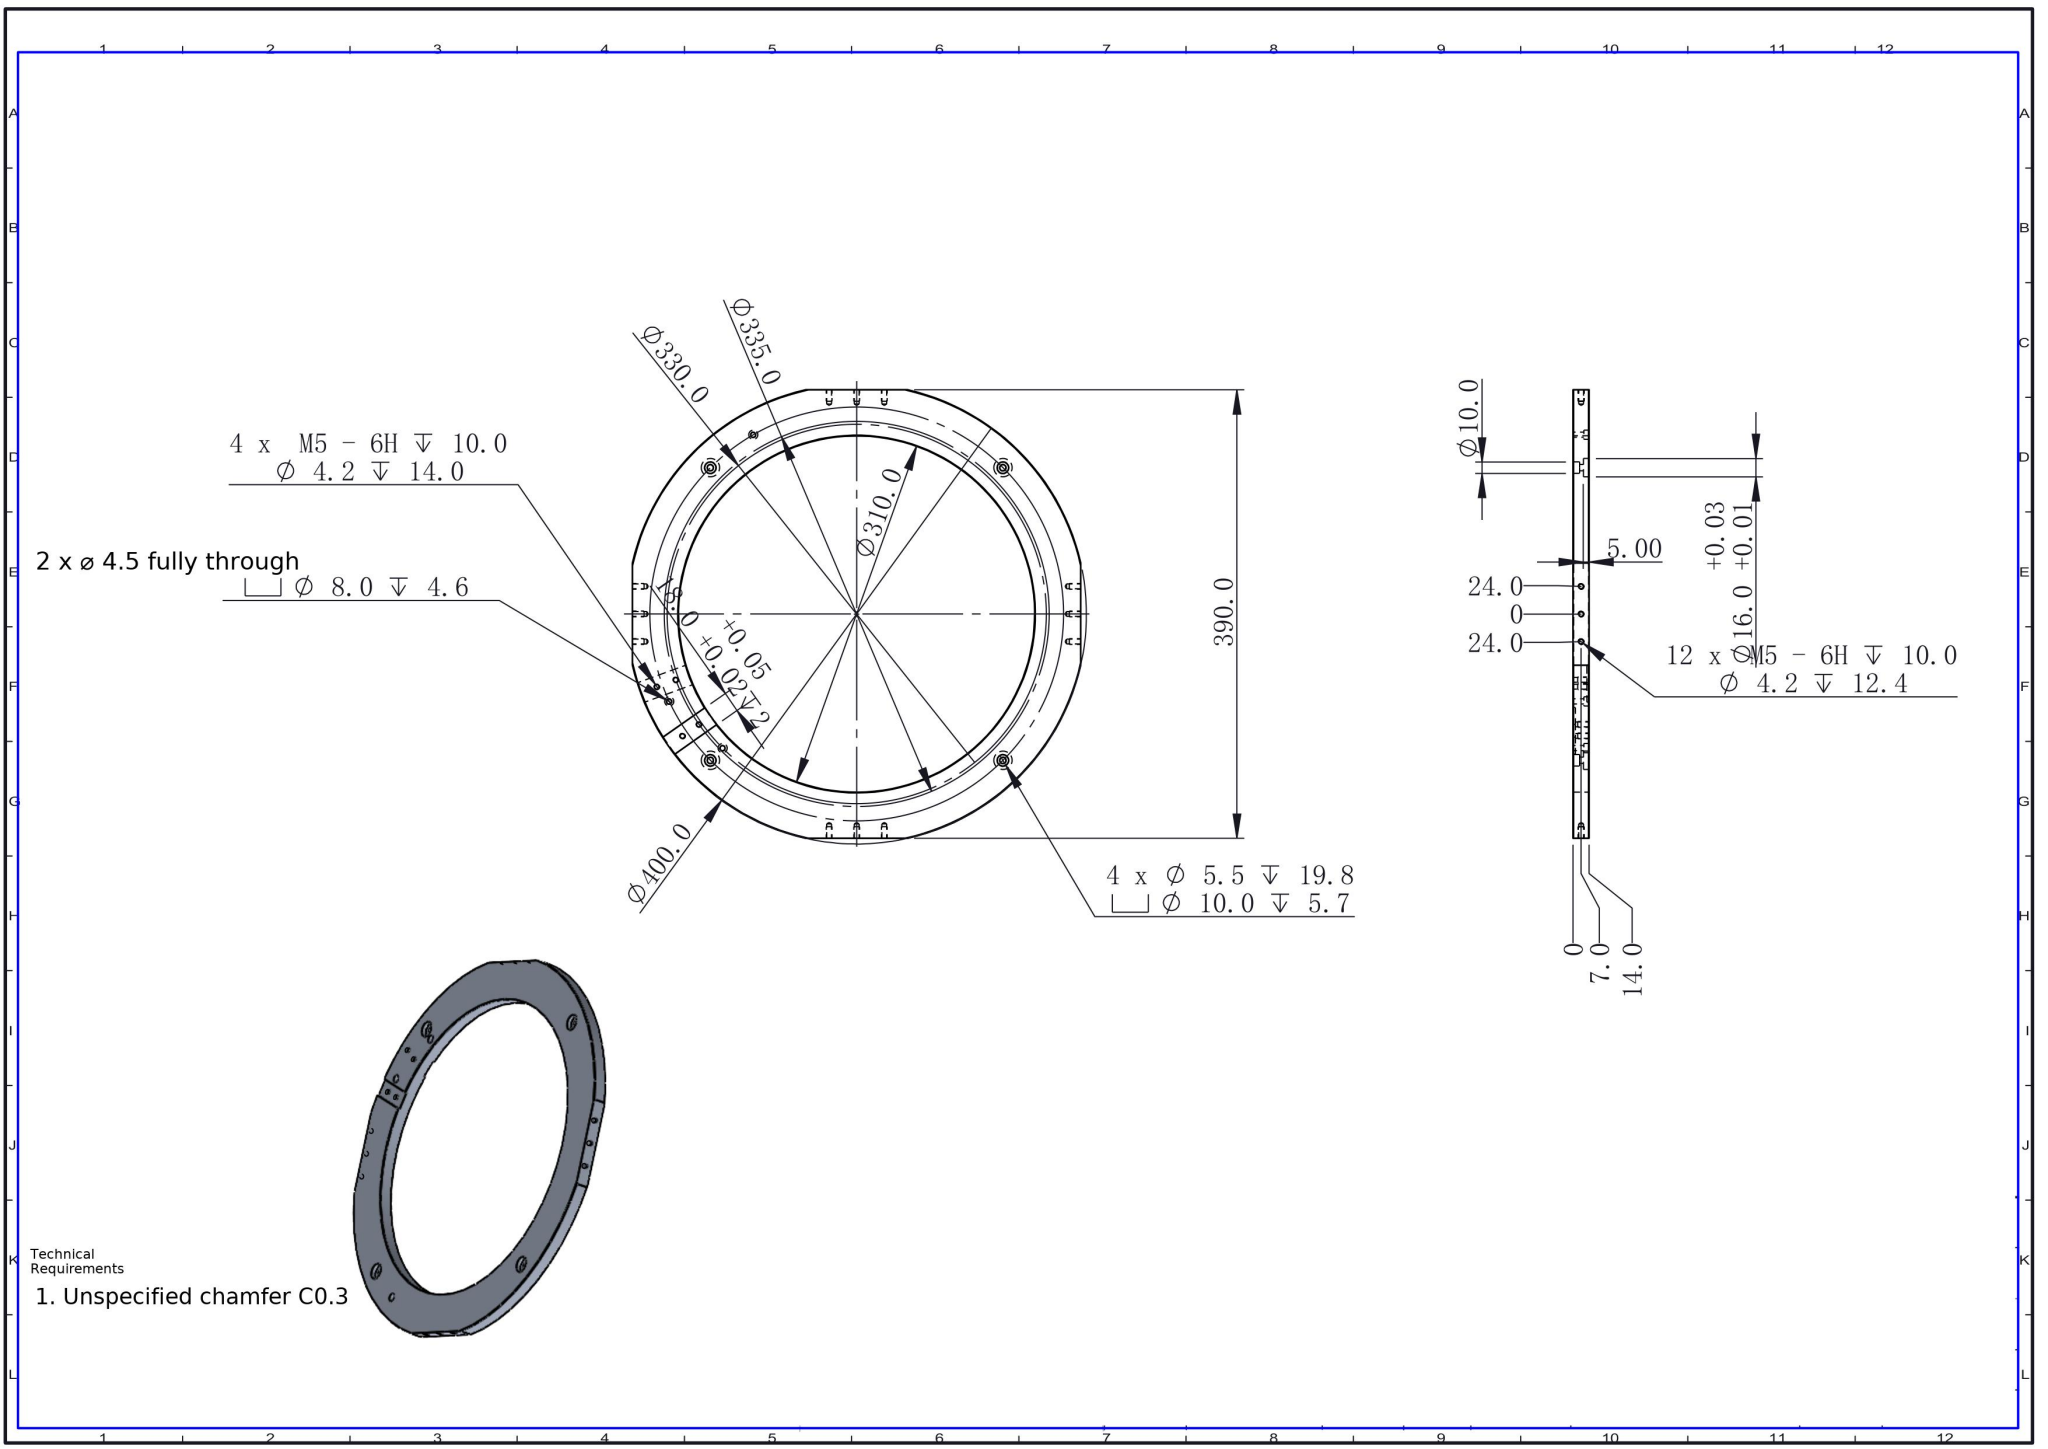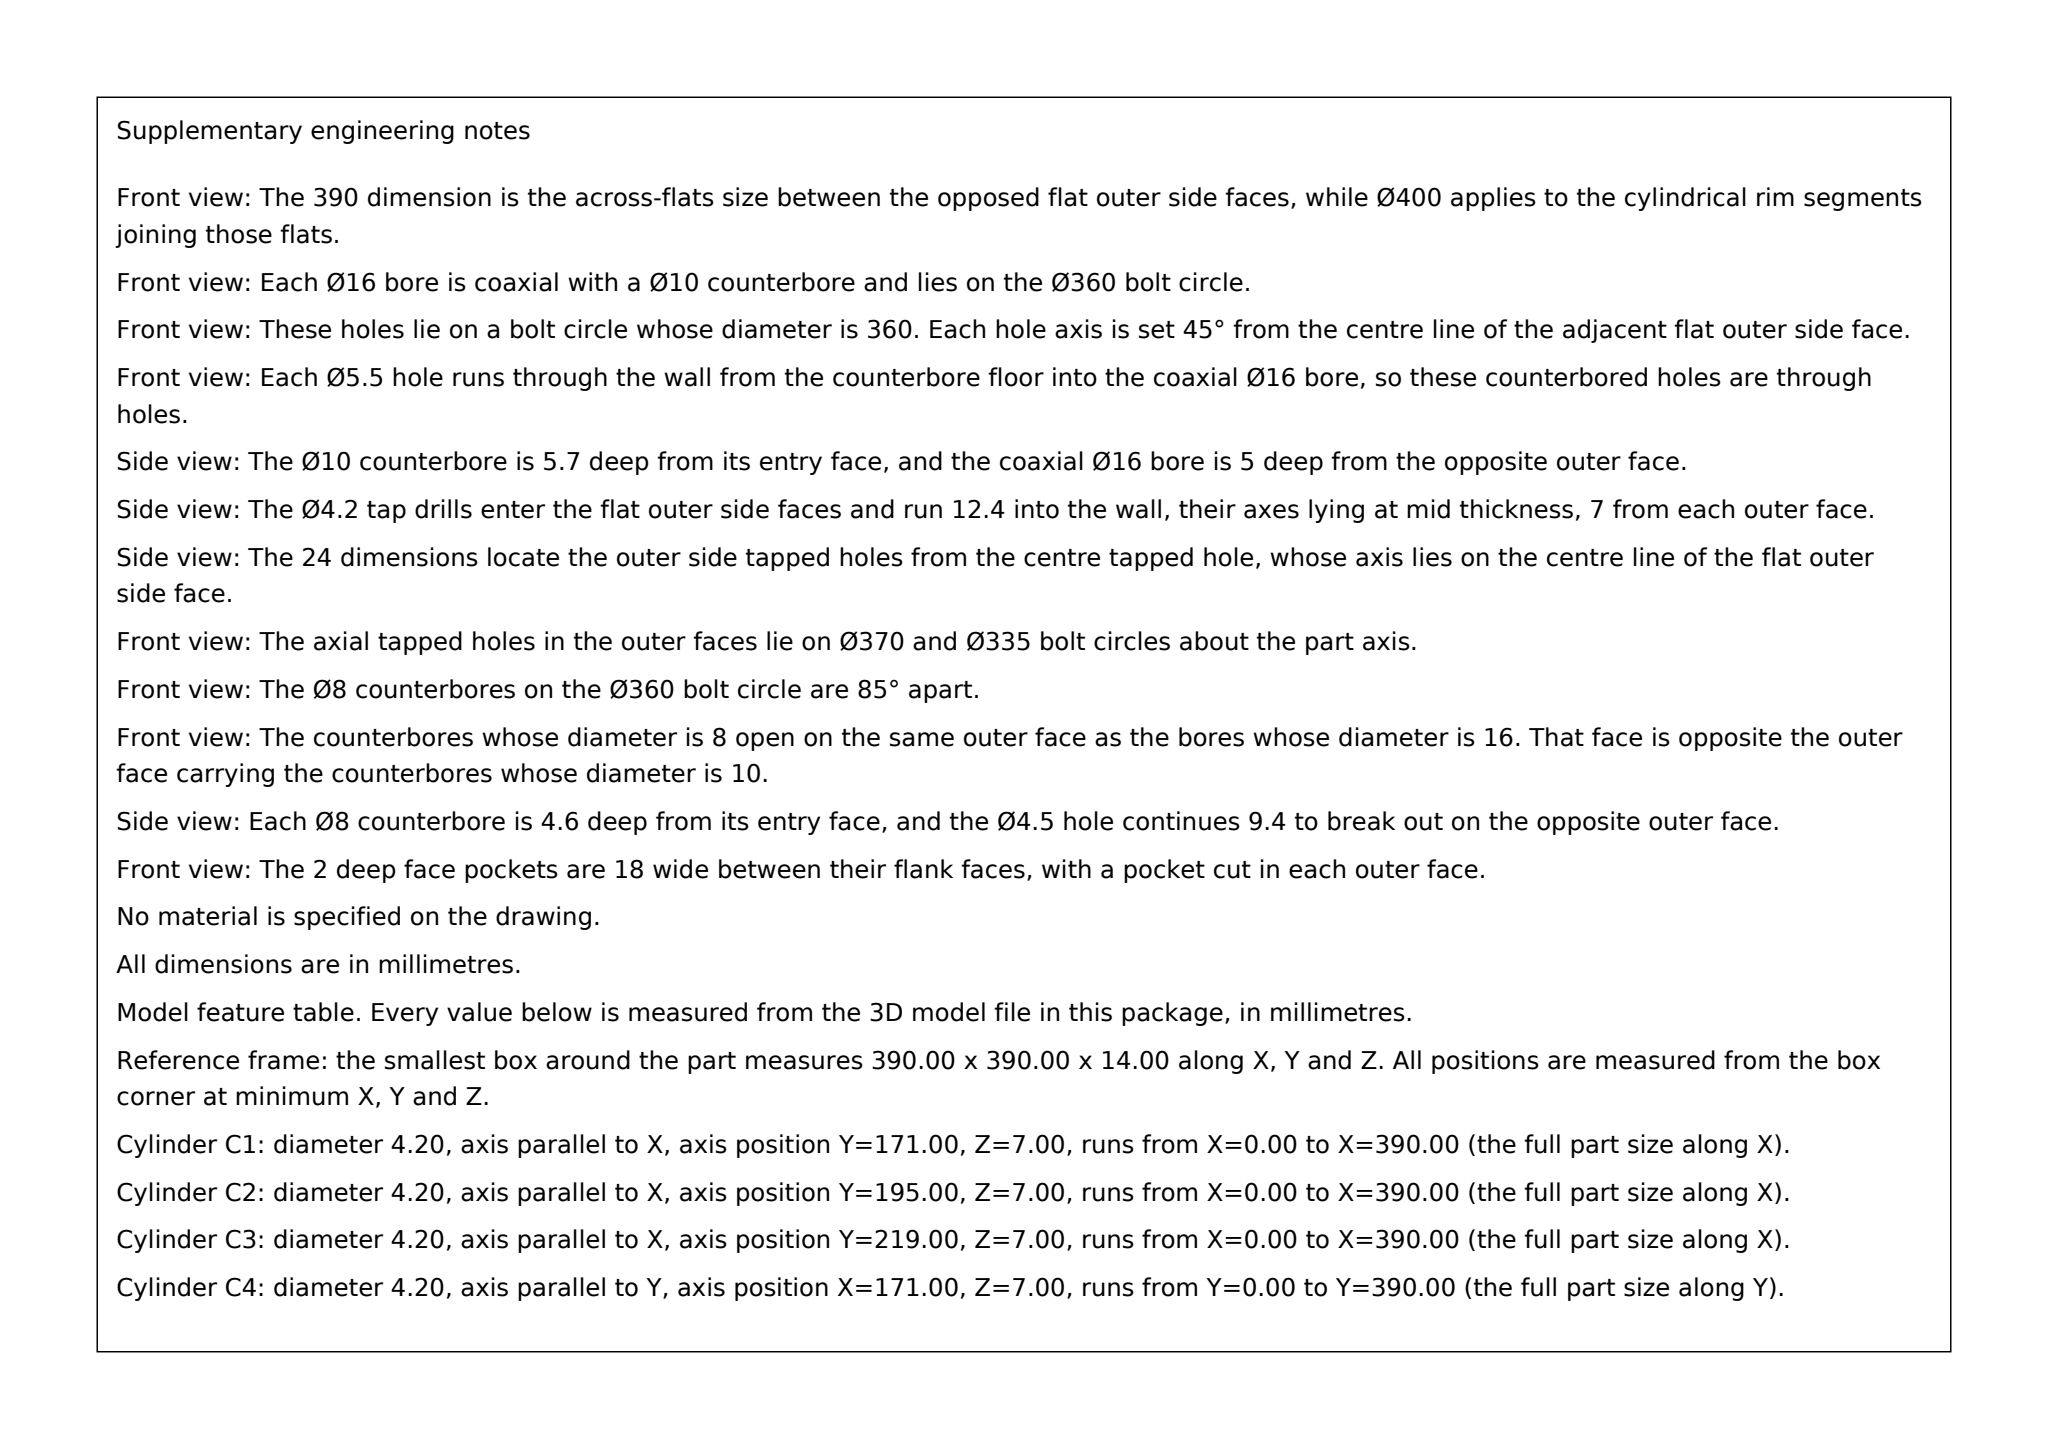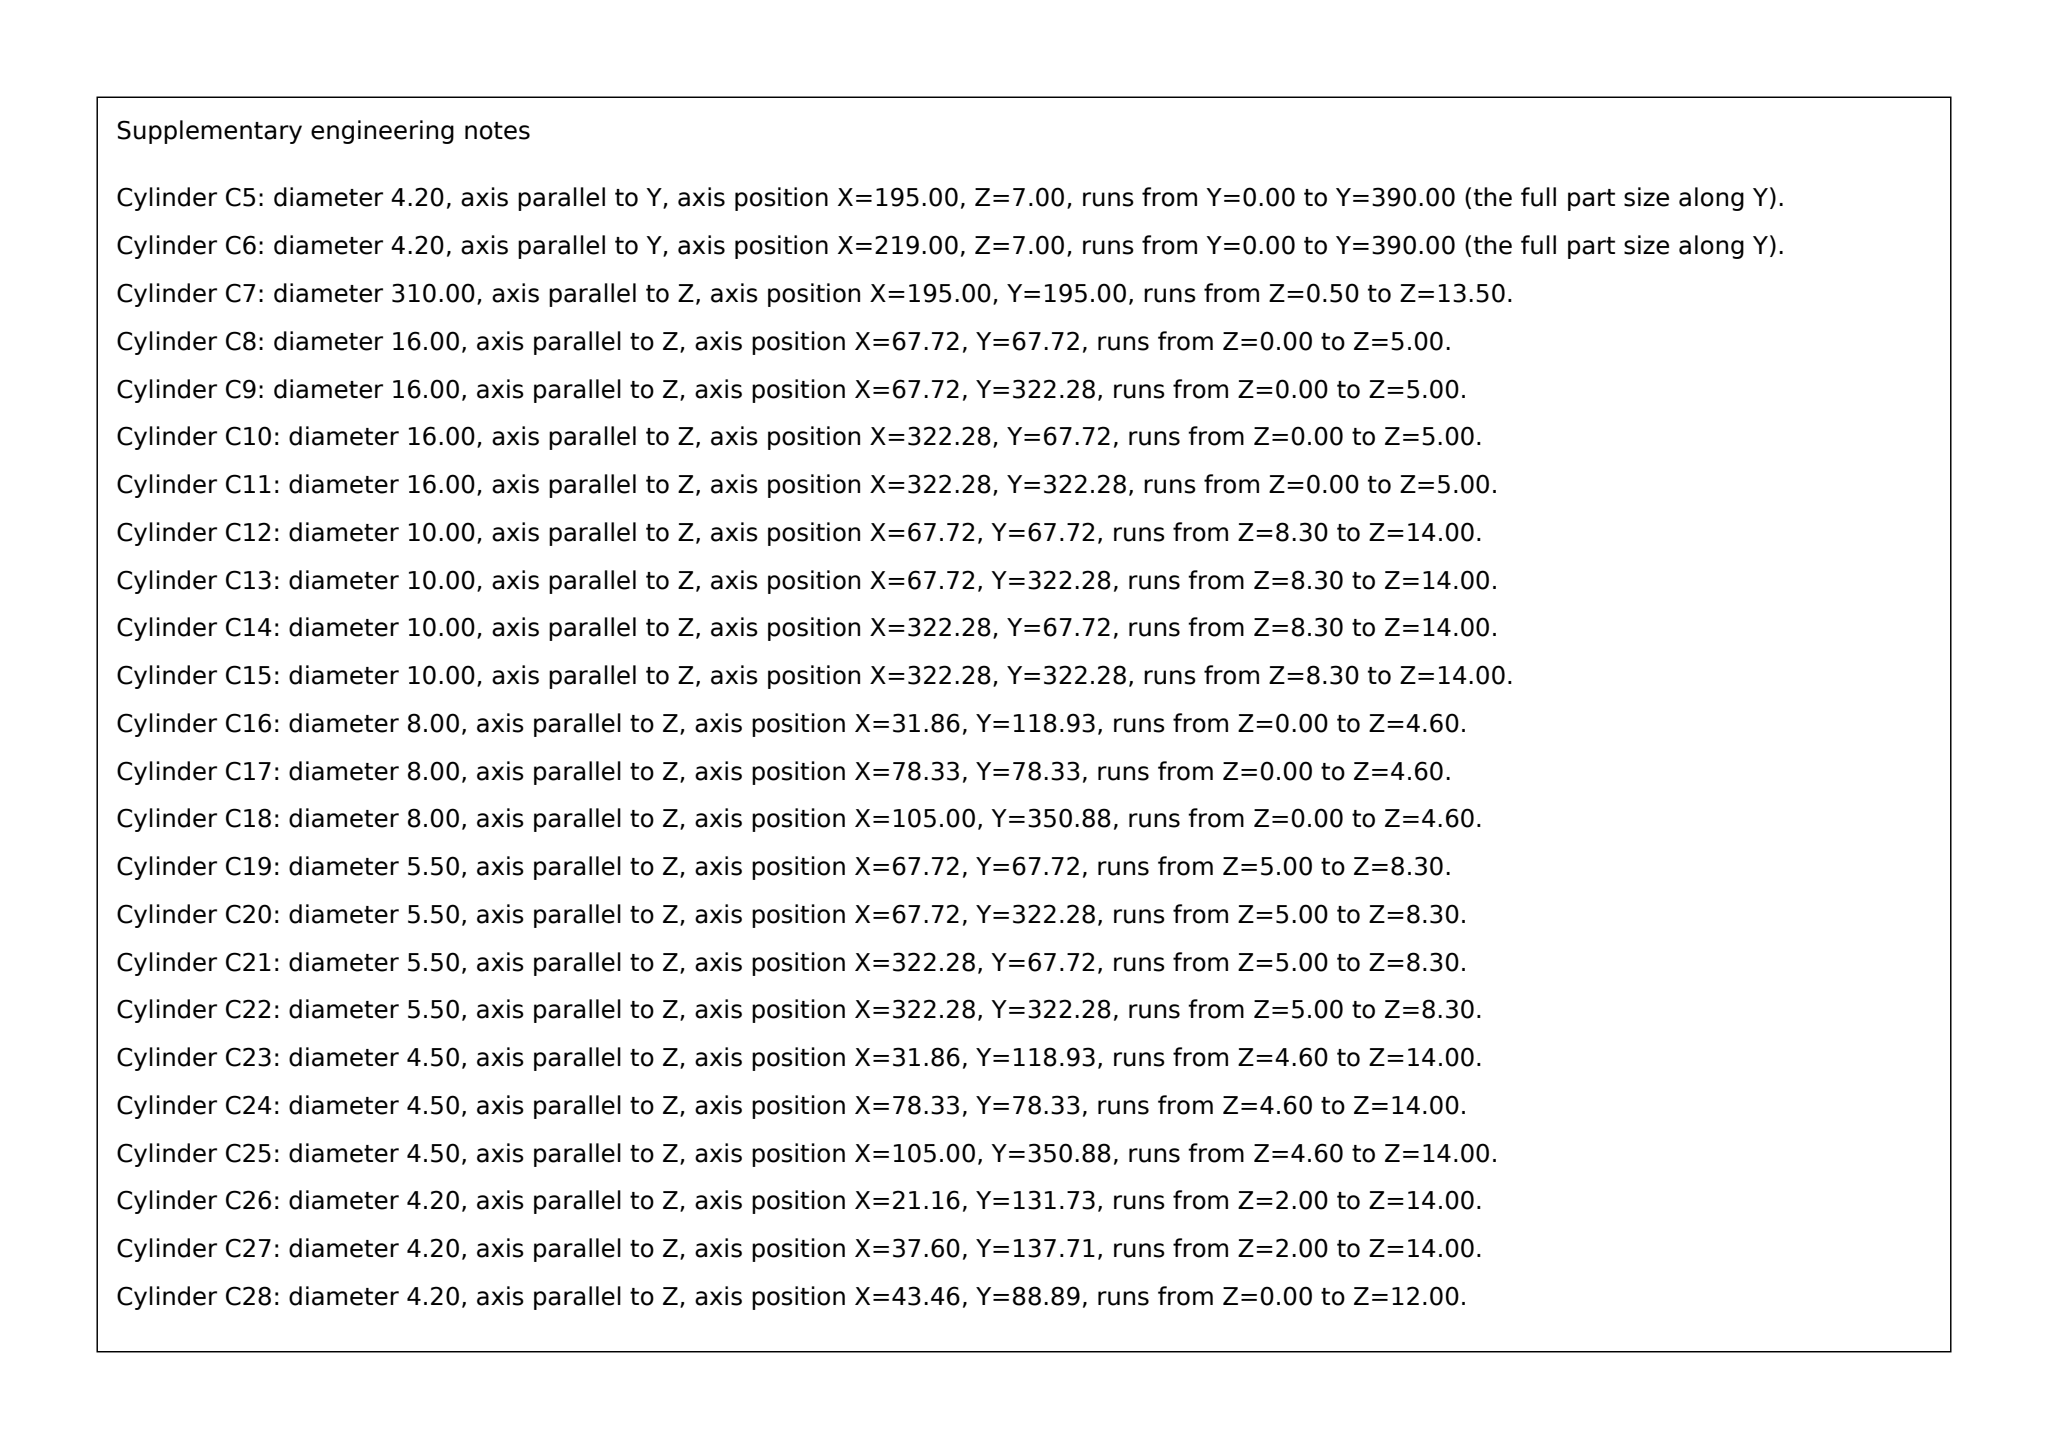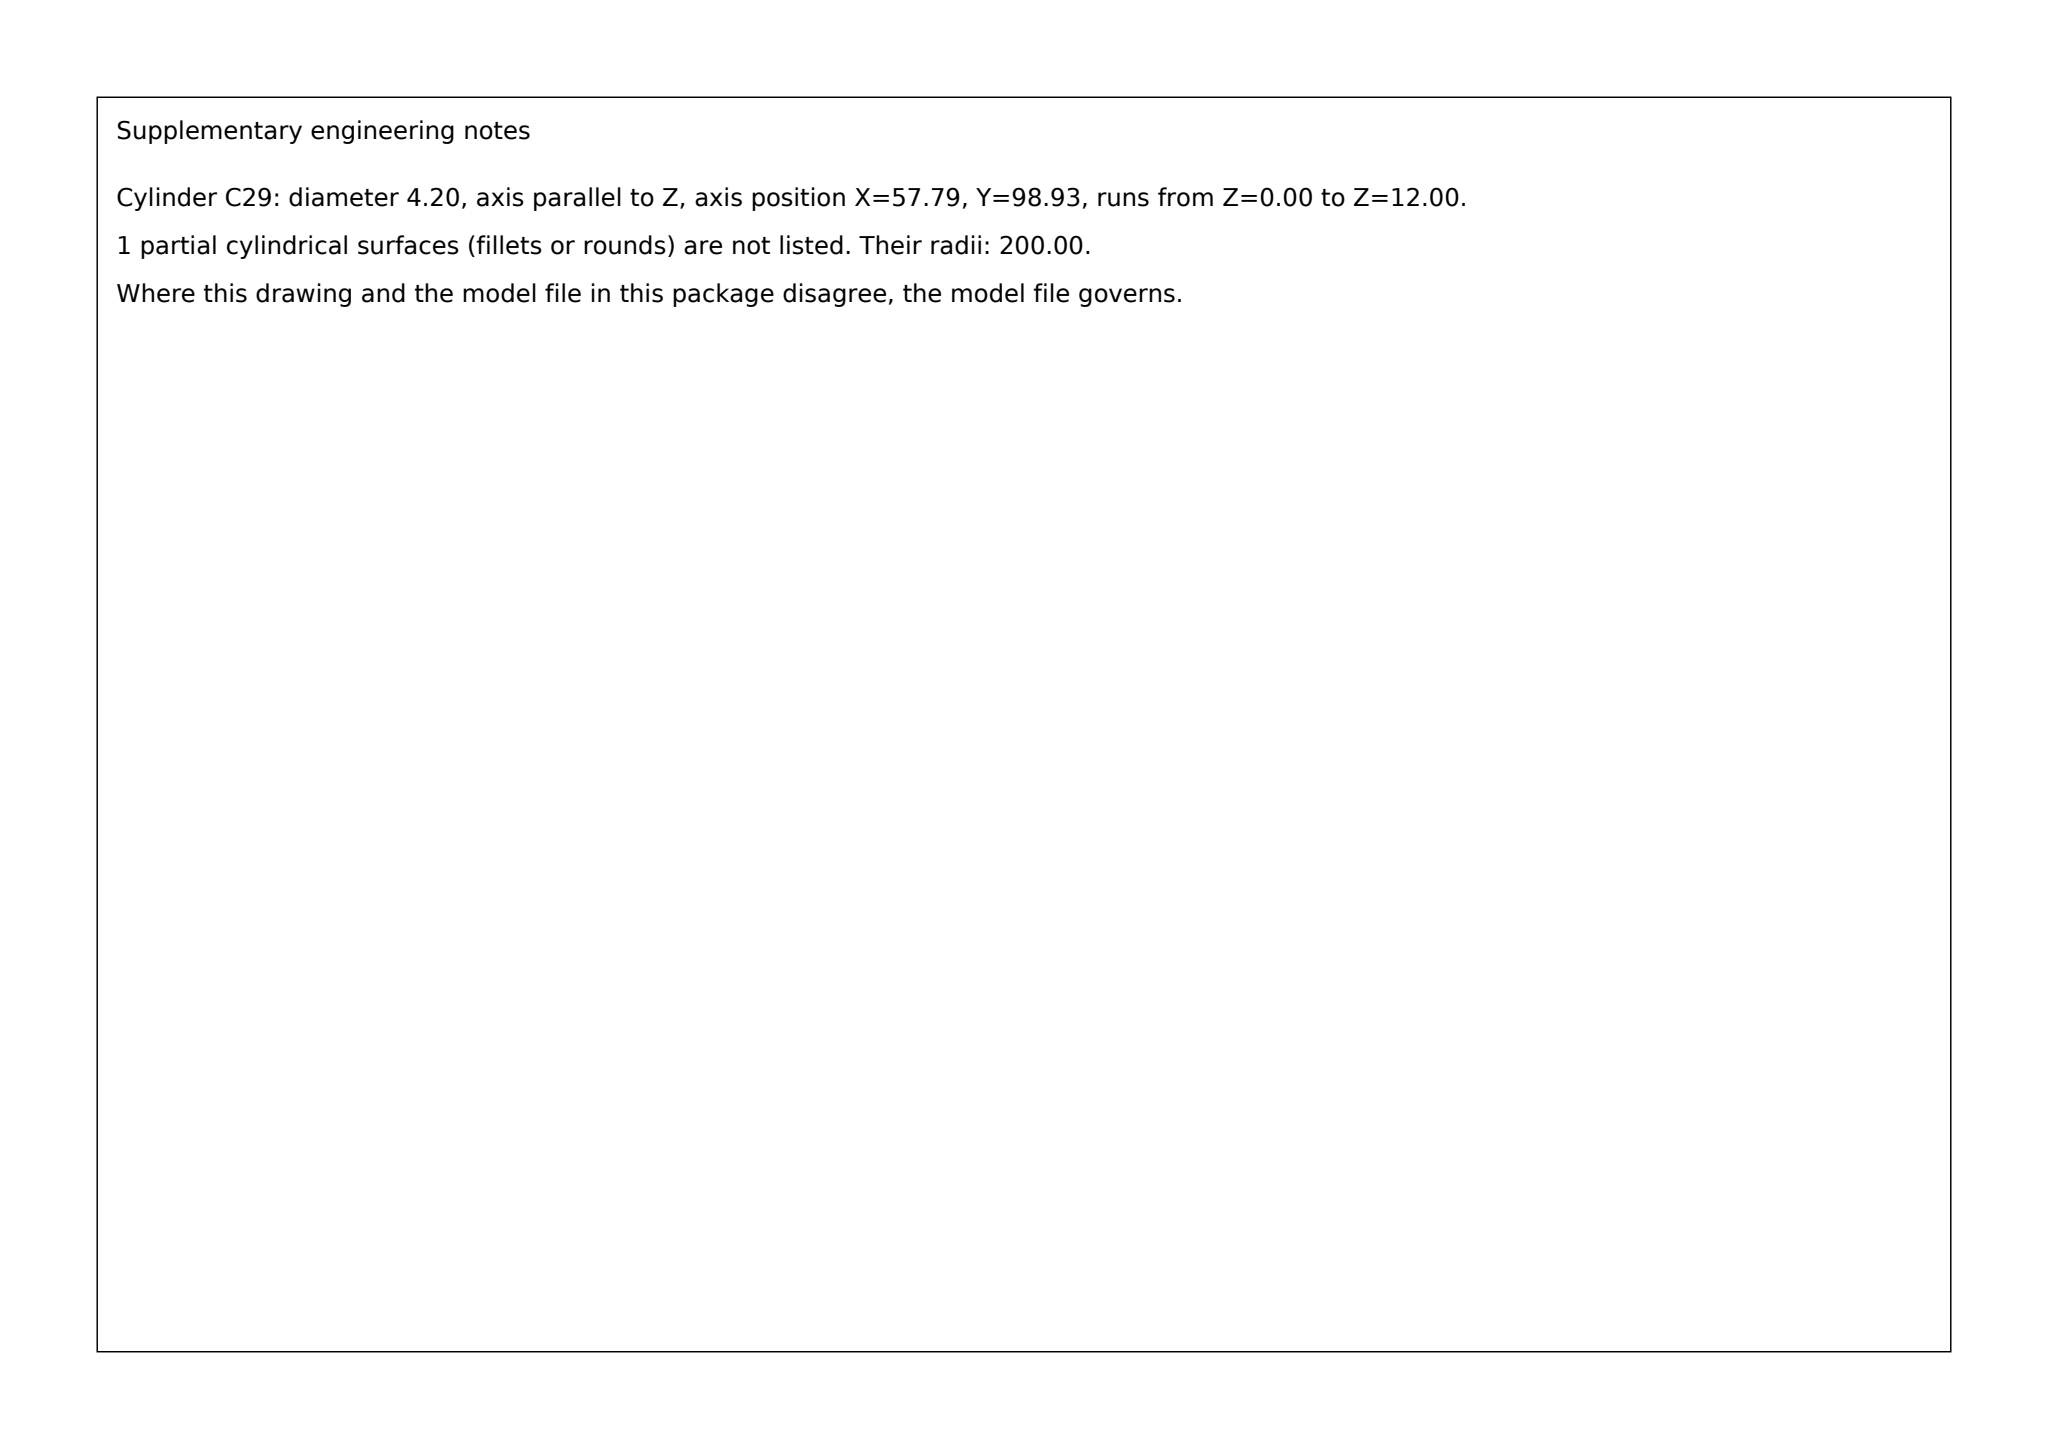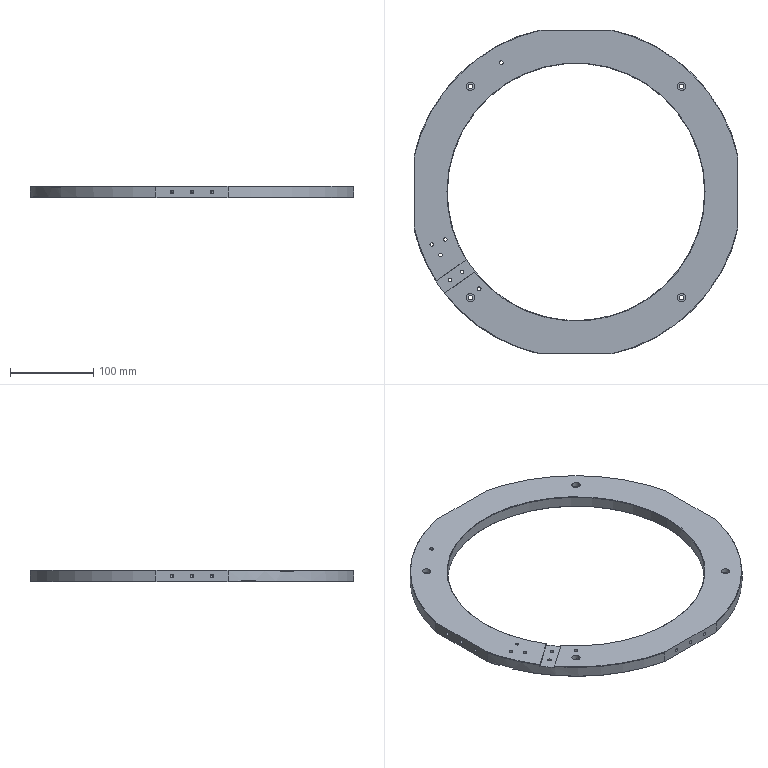Part | SolidWorks | mm | 1 solid | 137 faces | box 390 x 390 x 14 mm | volume 672218 mm3 | cylinder 74 | cone 40 | plane 23 | commonest cylinder face diameters 4.2 x32 10 x8 5.5 x8 16 x8 8 x6 4.5 x6 400 x4 310 x2
Drawing notes:
All dimensions in millimetres unless stated. | from the solid: STEP model units: mm
3X Ø4.5 THRU, CBORE Ø8.0 ▽4.6 from datum A (face z=0); located 60.0° above left horiz. CL on Ø360.0 B.C., 25.0° below left horiz. CL on Ø360.0 B.C., and 45.0° below left horiz. CL on Ø330.0 B.C. | from the solid: cylinders Ø4.5 z at (32.35,119.42),(78.82,78.82),(105.49,351.37) L9.4 and Ø8.0 z L4.6; centre 195.49,195.49; axis_planes z 4.6
4X M5 axial tapped holes: 2 on Ø370.0 B.C. (20.0° and 35.0° below left horiz. CL) and 2 on Ø335.0 B.C. (20.0° and 35.0° below left horiz. CL). | from the solid: cylinders Ø4.2 z at (21.65,132.21),(43.95,89.38) → R185.0; (38.09,138.2),(58.28,99.41) → R167.5 from centre 195.49,195.49
Ring OD: Ø390.98 arc, cut by four flats 195.0 from the centre axis (390.0 across flats), flats normal to the X and Y centrelines, 90° apart; flat chord width 27.7. | from the solid: bbox_xyz 390.977 sq; axis_planes x 0.49/390.49, y 0.49/390.49; centre 195.49,195.49
12X M5-6H ▽10.0 / Ø4.2 ▽12.4 radial tapped holes, 3 per OD flat on the X and Y centrelines (90° apart), at 0 and ±24.0 from the flat centre, axes 7.0 from datum A. | from the solid: cylinders Ø4.2 axis x at y=171.49/195.49/219.49 z=7.0 L12.4 and axis y at x=171.49/195.49/219.49 z=7.0 L12.4
4X Ø5.5 ▽19.8 holes equally spaced on Ø360.0 B.C., one per quadrant at 45.0° to the X/Y centrelines. | from the solid: cylinders Ø5.5 z at (68.21,68.21),(68.21,322.77),(322.77,68.21),(322.77,322.77); R180.0 at 45° from centre 195.49,195.49
Counterbore sides for the Ø5.5 holes: CBORE Ø16.0(+0.03/+0.01) ▽5.0 from datum A (z=0 face); CBORE Ø10.0 ▽5.7 from the opposite face (z=14.0). | from the solid: cylinders Ø16.0 z L5.0 with axis_plane z 5.0 (x4); cylinders Ø10.0 z L5.7 with axis_plane z 8.3 (x4); thickness 14.0
Datum A = face at z=0 (face carrying the Ø16.0 counterbores). The 4X M5 axial taps (drill 12.0 deep) and the 3X CBORE Ø8.0 ▽4.6 counterbores are machined from datum A. | from the solid: cylinders Ø4.2 z L12.0 with axis_plane z 12.0; Ø8.0 z L4.6 with axis_plane z 4.6; bbox thickness 14.0
Chamfer 0.5 x 45° on Ø310.0 bore and on the OD, both faces; this supersedes the C0.3 general note for these edges. | from the solid: cones 90° ref dia 310.0/311.0 (x3) and 400.0/399.0 (x5)
build123d program:
from build123d import *

# Parameters (mm, degrees)
SKETCH1_R                                         = 200
SKETCH1_R_2                                       = 155
BOSS_EXTRUDE1_DEPTH                               = 7
CHAMFER1_SIZE                                     = 0.5
SKETCH9_W                                         = 88.882
SKETCH9_H                                         = 146.064
SKETCH9_W_2                                       = 146.064
SKETCH9_H_2                                       = 88.882
CUT_EXTRUDE4_DEPTH                                = 14
M5_TAPPED_HOLE1_AT_2_COUNT                        = 2
M5_TAPPED_HOLE1_AT_2_PITCH                        = 24
M5_TAPPED_HOLE1_AT_3_COUNT                        = 2
M5_TAPPED_HOLE1_AT_3_PITCH                        = 48
CIRPATTERN1_COUNT                                 = 4
SKETCH12_R                                        = 8
CUT_EXTRUDE5_DEPTH                                = 5
HOLE_SIZE_ACCORDING_TO_TYPE_3_OF_HEXA_D           = 5.5
HOLE_SIZE_ACCORDING_TO_TYPE_3_OF_HEXA_DEPTH       = 19.8
HOLE_SIZE_ACCORDING_TO_TYPE_3_OF_HEXA_CBORE_D     = 10
HOLE_SIZE_ACCORDING_TO_TYPE_3_OF_HEXA_CBORE_DEPTH = 5.7
HOLE_SIZE_ACCORDING_TO_TYPE_3_OF_HEXA_TIP         = 1.652
HOLE_SIZE_ACCORDING_TO_TYPE_1_OF_HEXA_D           = 4.5
HOLE_SIZE_ACCORDING_TO_TYPE_1_OF_HEXA_CBORE_D     = 8
HOLE_SIZE_ACCORDING_TO_TYPE_1_OF_HEXA_CBORE_DEPTH = 4.6
CUT_EXTRUDE6_DEPTH                                = 2
HOLE_SIZE_ACCORDING_TO_TYPE_3_OF_2_D              = 4.5
HOLE_SIZE_ACCORDING_TO_TYPE_3_OF_2_CBORE_D        = 8
HOLE_SIZE_ACCORDING_TO_TYPE_3_OF_2_CBORE_DEPTH    = 4.6
CUT_EXTRUDE7_DEPTH                                = 2
M5_TAPPED_HOLE2_D                                 = 4.2
M5_TAPPED_HOLE2_DEPTH                             = 14
M5_TAPPED_HOLE2_TIP                               = 1.262


with BuildPart() as part:
    # Sketch1 → Boss-Extrude1 (new, symmetric)
    with BuildSketch(Plane.XY):
        Circle(SKETCH1_R)
        Circle(SKETCH1_R_2, mode=Mode.SUBTRACT)
    extrude(amount=BOSS_EXTRUDE1_DEPTH, both=True)

    # Chamfer1
    chamfer1_edges = [part.edges().sort_by_distance(p)[0] for p in [
        (-200, 0, -7),
        (-200, 0, 7),
        (-155, 0, -7),
        (-155, 0, 7),
    ]]
    chamfer(chamfer1_edges, length=CHAMFER1_SIZE)

    # Sketch9 → Cut-Extrude4 (cut)
    with BuildSketch(Plane(origin=(0, 0, -7), x_dir=(-1, 0, 0), z_dir=(0, 0, -1))):
        with Locations((0, -268.032)):
            Rectangle(SKETCH9_W, SKETCH9_H)
        with Locations((268.032, 0)):
            Rectangle(SKETCH9_W_2, SKETCH9_H_2)
        with Locations((-268.032, 0)):
            Rectangle(SKETCH9_W_2, SKETCH9_H_2)
        with Locations((0, 268.032)):
            Rectangle(SKETCH9_W, SKETCH9_H)
    extrude(amount=-CUT_EXTRUDE4_DEPTH, mode=Mode.SUBTRACT)

    # Sketch11 → M5 Tapped Hole1 (revolve, cut)
    with BuildSketch(Plane(origin=(-195, 24, 0), x_dir=(0, 0, 1), z_dir=(0, 1, 0))):
        Polygon((0, 0), (0, 13.662), (2.1, 12.4), (2.1, 0), align=None)
    m5_tapped_hole1 = revolve(axis=Axis((-201.35, 24, 0), (1, 0, 0)), mode=Mode.SUBTRACT)

    # M5 Tapped Hole1 at 2: M5 Tapped Hole1 ×2
    with Locations(*[(0, -i * M5_TAPPED_HOLE1_AT_2_PITCH, 0) for i in range(1, M5_TAPPED_HOLE1_AT_2_COUNT)]):
        add(m5_tapped_hole1, mode=Mode.SUBTRACT)

    # M5 Tapped Hole1 at 3: M5 Tapped Hole1 ×2
    with Locations(*[(0, -i * M5_TAPPED_HOLE1_AT_3_PITCH, 0) for i in range(1, M5_TAPPED_HOLE1_AT_3_COUNT)]):
        add(m5_tapped_hole1, mode=Mode.SUBTRACT)

    # CirPattern1: M5 Tapped Hole1 ×4 about axis
    cirpattern1_axis = Axis((0, 0, 7), (0, 0, -1))
    for i in range(1, CIRPATTERN1_COUNT):
        add(m5_tapped_hole1.rotate(cirpattern1_axis, i * 360 / CIRPATTERN1_COUNT), mode=Mode.SUBTRACT)

    # CirPattern1 copy 1 sketch → CirPattern1 copy 1 (revolve, cut)
    with BuildSketch(Plane(origin=(0, 195, 0), x_dir=(0, 0, 1), z_dir=(1, 0, 0))):
        Polygon((0, 0), (0, 13.662), (2.1, 12.4), (2.1, 0), align=None)
    revolve(axis=Axis((0, 201.35, 0), (0, -1, 0)), mode=Mode.SUBTRACT)

    # CirPattern1 copy 2 sketch → CirPattern1 copy 2 (revolve, cut)
    with BuildSketch(Plane(origin=(195, 0, 0), x_dir=(0, 0, 1), z_dir=(0, -1, 0))):
        Polygon((0, 0), (0, 13.662), (2.1, 12.4), (2.1, 0), align=None)
    revolve(axis=Axis((201.35, 0, 0), (-1, 0, 0)), mode=Mode.SUBTRACT)

    # CirPattern1 copy 3 sketch → CirPattern1 copy 3 (revolve, cut)
    with BuildSketch(Plane(origin=(0, -195, 0), x_dir=(0, 0, 1), z_dir=(-1, 0, 0))):
        Polygon((0, 0), (0, 13.662), (2.1, 12.4), (2.1, 0), align=None)
    revolve(axis=Axis((0, -201.35, 0), (0, 1, 0)), mode=Mode.SUBTRACT)

    # CirPattern1 copy 4 sketch → CirPattern1 copy 4 (revolve, cut)
    with BuildSketch(Plane(origin=(-24, 195, 0), x_dir=(0, 0, 1), z_dir=(1, 0, 0))):
        Polygon((0, 0), (0, 13.662), (2.1, 12.4), (2.1, 0), align=None)
    revolve(axis=Axis((-24, 201.35, 0), (0, -1, 0)), mode=Mode.SUBTRACT)

    # CirPattern1 copy 5 sketch → CirPattern1 copy 5 (revolve, cut)
    with BuildSketch(Plane(origin=(195, 24, 0), x_dir=(0, 0, 1), z_dir=(0, -1, 0))):
        Polygon((0, 0), (0, 13.662), (2.1, 12.4), (2.1, 0), align=None)
    revolve(axis=Axis((201.35, 24, 0), (-1, 0, 0)), mode=Mode.SUBTRACT)

    # CirPattern1 copy 6 sketch → CirPattern1 copy 6 (revolve, cut)
    with BuildSketch(Plane(origin=(24, -195, 0), x_dir=(0, 0, 1), z_dir=(-1, 0, 0))):
        Polygon((0, 0), (0, 13.662), (2.1, 12.4), (2.1, 0), align=None)
    revolve(axis=Axis((24, -201.35, 0), (0, 1, 0)), mode=Mode.SUBTRACT)

    # Sketch12 → Cut-Extrude5 (cut)
    with BuildSketch(Plane(origin=(0, 0, -7), x_dir=(-1, 0, 0), z_dir=(0, 0, -1))):
        with Locations((127.279, 127.279)):
            Circle(SKETCH12_R)
        with Locations((127.279, -127.279)):
            Circle(SKETCH12_R)
        with Locations((-127.279, -127.279)):
            Circle(SKETCH12_R)
        with Locations((-127.279, 127.279)):
            Circle(SKETCH12_R)
    extrude(amount=-CUT_EXTRUDE5_DEPTH, mode=Mode.SUBTRACT)

    # Hole Size _ according to_ Type 3 of Hexa
    with Locations(Plane.XY.offset(7)):
        with Locations((127.279, -127.279), (-127.279, -127.279), (-127.279, 127.279), (127.279, 127.279)):
            CounterBoreHole(HOLE_SIZE_ACCORDING_TO_TYPE_3_OF_HEXA_D / 2, HOLE_SIZE_ACCORDING_TO_TYPE_3_OF_HEXA_CBORE_D / 2, HOLE_SIZE_ACCORDING_TO_TYPE_3_OF_HEXA_CBORE_DEPTH, depth=HOLE_SIZE_ACCORDING_TO_TYPE_3_OF_HEXA_DEPTH)
            with Locations((0, 0, -(HOLE_SIZE_ACCORDING_TO_TYPE_3_OF_HEXA_DEPTH + HOLE_SIZE_ACCORDING_TO_TYPE_3_OF_HEXA_TIP / 2))):  # 118° drill point
                Cone(0, HOLE_SIZE_ACCORDING_TO_TYPE_3_OF_HEXA_D / 2, HOLE_SIZE_ACCORDING_TO_TYPE_3_OF_HEXA_TIP, mode=Mode.SUBTRACT)

    # Hole Size _ according to_ Type 1 of Hexa (through all)
    with Locations(Plane(origin=(0, 0, -7), x_dir=(1, 0, 0), z_dir=(0, 0, -1))):
        with Locations((-90, -155.885), (-163.135, 76.071)):
            CounterBoreHole(HOLE_SIZE_ACCORDING_TO_TYPE_1_OF_HEXA_D / 2, HOLE_SIZE_ACCORDING_TO_TYPE_1_OF_HEXA_CBORE_D / 2, HOLE_SIZE_ACCORDING_TO_TYPE_1_OF_HEXA_CBORE_DEPTH)

    # Sketch23 → Cut-Extrude6 (cut)
    with BuildSketch(Plane.XY.offset(7)):
        Polygon((-54.248, -48.972), (-255.412, -189.829), (-265.737, -175.084), (-64.573, -34.227), align=None)
    extrude(amount=-CUT_EXTRUDE6_DEPTH, mode=Mode.SUBTRACT)

    # Hole Size _ according to_ Type 3 of  2 (through all)
    with Locations(Plane(origin=(0, 0, -7), x_dir=(1, 0, 0), z_dir=(0, 0, -1))):
        with Locations((-116.673, 116.673)):
            CounterBoreHole(HOLE_SIZE_ACCORDING_TO_TYPE_3_OF_2_D / 2, HOLE_SIZE_ACCORDING_TO_TYPE_3_OF_2_CBORE_D / 2, HOLE_SIZE_ACCORDING_TO_TYPE_3_OF_2_CBORE_DEPTH)

    # Sketch26 → Cut-Extrude7 (cut)
    with BuildSketch(Plane(origin=(0, 0, -7), x_dir=(-1, 0, 0), z_dir=(0, 0, -1))):
        Polygon((98.982, -45.604), (105.138, -28.689), (308.427, -102.681), (302.27, -119.595), align=None)
    extrude(amount=-CUT_EXTRUDE7_DEPTH, mode=Mode.SUBTRACT)

    # M5 Tapped Hole2
    with Locations(Plane(origin=(0, 0, -7), x_dir=(-1, 0, 0), z_dir=(0, 0, -1))):
        with Locations((173.843, -63.274), (157.399, -57.288), (137.208, -96.074), (151.543, -106.112)):
            Hole(M5_TAPPED_HOLE2_D / 2, depth=M5_TAPPED_HOLE2_DEPTH)
            with Locations((0, 0, -(M5_TAPPED_HOLE2_DEPTH + M5_TAPPED_HOLE2_TIP / 2))):  # 118° drill point
                Cone(0, M5_TAPPED_HOLE2_D / 2, M5_TAPPED_HOLE2_TIP, mode=Mode.SUBTRACT)


solid = part.part